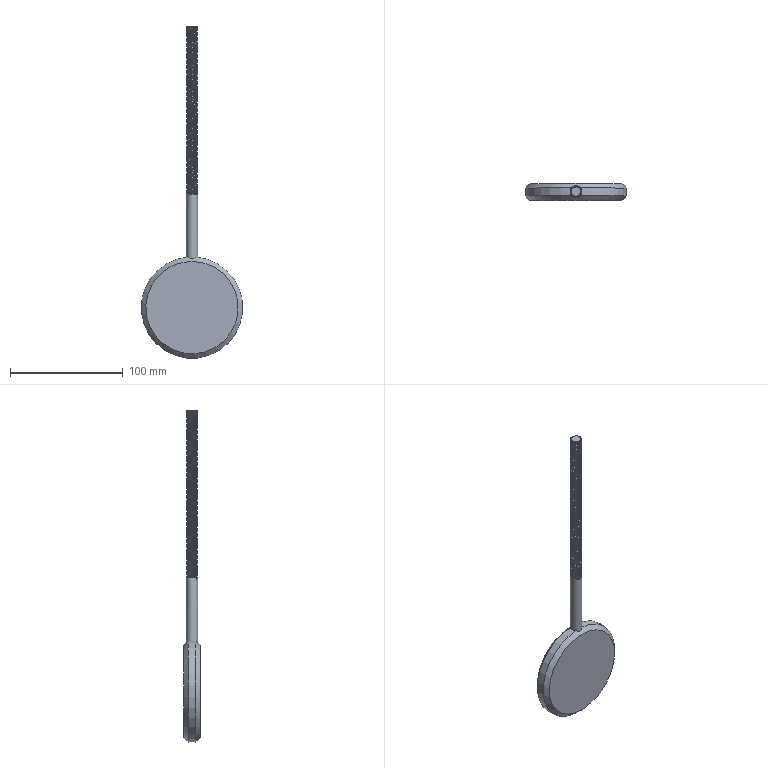Component | NX | VALVE_CAP | 1 solid | 110 faces | volume 103268 mm3 | cylinder 102 | plane 4 | cone 2 | spline 2 | commonest cylinder face diameters 10 x100 90 x1 8.5 x1